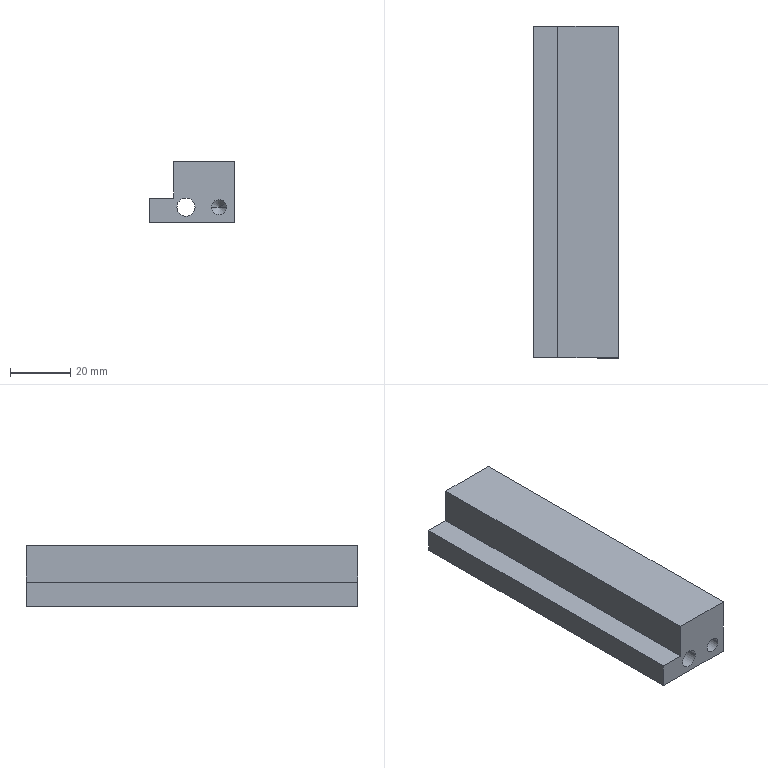Component | SolidWorks | OuterBagSealingCopperBlock-1 | 1 solid | 22 faces | box 28 x 110 x 20 mm | volume 47407 mm3 | cylinder 8 | plane 8 | cone 6 | commonest cylinder face diameters 3.3 x4 5 x2 6 x2
build123d program:
from build123d import *

# Parameters (mm, degrees)
BOSS_EXTRUDE1_DEPTH   = 55
M4_TAPPED_HOLE1_D     = 3.3
M4_TAPPED_HOLE1_DEPTH = 12.1
M4_TAPPED_HOLE1_TIP   = 0.9526
SKETCH4_R             = 3
CUT_EXTRUDE1_DEPTH    = 110
M6_TAPPED_HOLE1_D     = 5
M6_TAPPED_HOLE1_DEPTH = 15
M6_TAPPED_HOLE1_TIP   = 2.5


with BuildPart() as part:
    # Sketch1 → Boss-Extrude1 (new, symmetric)
    with BuildSketch(Plane.XY):
        Polygon((0, 0), (0, 20), (28, 20), (28, 12), (20, 12), (20, 0), align=None)
    extrude(amount=BOSS_EXTRUDE1_DEPTH, both=True)

    # M4 Tapped Hole1
    with Locations(Plane(origin=(0, 10, -25), x_dir=(0, 0, -1), z_dir=(-1, 0, 0))):
        with Locations((0, 0), (-50, 0)):
            Hole(M4_TAPPED_HOLE1_D / 2, depth=M4_TAPPED_HOLE1_DEPTH)
            with Locations((0, 0, -(M4_TAPPED_HOLE1_DEPTH + M4_TAPPED_HOLE1_TIP / 2))):  # 120° drill point
                Cone(0, M4_TAPPED_HOLE1_D / 2, M4_TAPPED_HOLE1_TIP, mode=Mode.SUBTRACT)

    # Sketch4 → Cut-Extrude1 (cut)
    with BuildSketch(Plane.XY.offset(55)):
        with Locations((16, 15)):
            Circle(SKETCH4_R)
    extrude(amount=-CUT_EXTRUDE1_DEPTH, mode=Mode.SUBTRACT)

    # M6 Tapped Hole1
    with Locations(Plane(origin=(5, 15, 55), x_dir=(1, 0, 0), z_dir=(0, 0, 1))):
        with Locations((0, 0)):
            Hole(M6_TAPPED_HOLE1_D / 2, depth=M6_TAPPED_HOLE1_DEPTH)
            with Locations((0, 0, -(M6_TAPPED_HOLE1_DEPTH + M6_TAPPED_HOLE1_TIP / 2))):  # 90° drill point
                Cone(0, M6_TAPPED_HOLE1_D / 2, M6_TAPPED_HOLE1_TIP, mode=Mode.SUBTRACT)


solid = part.part

# Placed as in the assembly
solid = solid.moved(Location((-43.341, 37.185, -31.775), (90, 0, -180)))
STEP:
#1=CARTESIAN_POINT('',(-1.805,-0.1108,-1.842));
#2=VERTEX_POINT('',#1);
#3=CARTESIAN_POINT('',(-2.002,-0.1108,-1.842));
#4=VERTEX_POINT('',#3);
#5=CARTESIAN_POINT('',(-1.903,-0.1108,-1.842));
#6=DIRECTION('',(-0.,-1.,0.));
#7=DIRECTION('',(-1.,0.,0.));
#8=AXIS2_PLACEMENT_3D('',#5,#6,#7);
#9=CIRCLE('',#8,0.09843);
#10=EDGE_CURVE('',#2,#4,#9,.T.);
#11=ORIENTED_EDGE('',*,*,#10,.F.);
#12=CARTESIAN_POINT('',(-1.805,-0.7014,-1.842));
#13=VERTEX_POINT('',#12);
#14=CARTESIAN_POINT('',(-1.805,-0.7014,-1.842));
#15=DIRECTION('',(-0.,-1.,0.));
#16=VECTOR('',#15,39.37);
#17=LINE('',#14,#16);
#18=EDGE_CURVE('',#2,#13,#17,.T.);
#19=ORIENTED_EDGE('',*,*,#18,.T.);
#20=CARTESIAN_POINT('',(-2.002,-0.7014,-1.842));
#21=VERTEX_POINT('',#20);
#22=CARTESIAN_POINT('',(-1.903,-0.7014,-1.842));
#23=DIRECTION('',(-0.,-1.,0.));
#24=DIRECTION('',(-1.,0.,0.));
#25=AXIS2_PLACEMENT_3D('',#22,#23,#24);
#26=CIRCLE('',#25,0.09843);
#27=EDGE_CURVE('',#13,#21,#26,.T.);
#28=ORIENTED_EDGE('',*,*,#27,.T.);
#29=CARTESIAN_POINT('',(-2.002,-0.7014,-1.842));
#30=DIRECTION('',(-0.,-1.,0.));
#31=VECTOR('',#30,39.37);
#32=LINE('',#29,#31);
#33=EDGE_CURVE('',#4,#21,#32,.T.);
#34=ORIENTED_EDGE('',*,*,#33,.F.);
#35=EDGE_LOOP('',(#11,#19,#28,#34));
#36=FACE_OUTER_BOUND('',#35,.T.);
#37=CARTESIAN_POINT('',(-1.903,-0.7014,-1.842));
#38=DIRECTION('',(-0.,-1.,0.));
#39=DIRECTION('',(-1.,0.,0.));
#40=AXIS2_PLACEMENT_3D('',#37,#38,#39);
#41=CYLINDRICAL_SURFACE('',#40,0.09843);
#42=ADVANCED_FACE('',(#36),#41,.F.);
#43=CARTESIAN_POINT('',(-1.903,-0.01239,-1.842));
#44=VERTEX_POINT('',#43);
#45=CARTESIAN_POINT('',(-2.002,-0.1108,-1.842));
#46=DIRECTION('',(-0.7071,-0.7071,0.));
#47=VECTOR('',#46,39.37);
#48=LINE('',#45,#47);
#49=EDGE_CURVE('',#44,#4,#48,.T.);
#50=ORIENTED_EDGE('',*,*,#49,.F.);
#51=CARTESIAN_POINT('',(-1.805,-0.1108,-1.842));
#52=DIRECTION('',(0.7071,-0.7071,-0.));
#53=VECTOR('',#52,39.37);
#54=LINE('',#51,#53);
#55=EDGE_CURVE('',#44,#2,#54,.T.);
#56=ORIENTED_EDGE('',*,*,#55,.T.);
#57=ORIENTED_EDGE('',*,*,#10,.T.);
#58=EDGE_LOOP('',(#50,#56,#57));
#59=FACE_OUTER_BOUND('',#58,.T.);
#60=CARTESIAN_POINT('',(-1.903,-0.1108,-1.842));
#61=DIRECTION('',(-0.,-1.,0.));
#62=DIRECTION('',(-1.,0.,0.));
#63=AXIS2_PLACEMENT_3D('',#60,#61,#62);
#64=CONICAL_SURFACE('',#63,0.09843,0.7854);
#65=ADVANCED_FACE('',(#59),#64,.F.);
#66=CARTESIAN_POINT('',(-2.218,3.629,-1.842));
#67=VERTEX_POINT('',#66);
#68=CARTESIAN_POINT('',(-2.454,3.629,-1.842));
#69=VERTEX_POINT('',#68);
#70=CARTESIAN_POINT('',(-2.336,3.629,-1.842));
#71=DIRECTION('',(-0.,-1.,0.));
#72=DIRECTION('',(-1.,0.,0.));
#73=AXIS2_PLACEMENT_3D('',#70,#71,#72);
#74=CIRCLE('',#73,0.1181);
#75=EDGE_CURVE('',#67,#69,#74,.T.);
#76=ORIENTED_EDGE('',*,*,#75,.F.);
#77=CARTESIAN_POINT('',(-2.218,-0.7014,-1.842));
#78=VERTEX_POINT('',#77);
#79=CARTESIAN_POINT('',(-2.218,3.629,-1.842));
#80=DIRECTION('',(-0.,-1.,0.));
#81=VECTOR('',#80,39.37);
#82=LINE('',#79,#81);
#83=EDGE_CURVE('',#67,#78,#82,.T.);
#84=ORIENTED_EDGE('',*,*,#83,.T.);
#85=CARTESIAN_POINT('',(-2.454,-0.7014,-1.842));
#86=VERTEX_POINT('',#85);
#87=CARTESIAN_POINT('',(-2.336,-0.7014,-1.842));
#88=DIRECTION('',(-0.,-1.,0.));
#89=DIRECTION('',(-1.,0.,0.));
#90=AXIS2_PLACEMENT_3D('',#87,#88,#89);
#91=CIRCLE('',#90,0.1181);
#92=EDGE_CURVE('',#78,#86,#91,.T.);
#93=ORIENTED_EDGE('',*,*,#92,.T.);
#94=CARTESIAN_POINT('',(-2.454,3.629,-1.842));
#95=DIRECTION('',(-0.,-1.,0.));
#96=VECTOR('',#95,39.37);
#97=LINE('',#94,#96);
#98=EDGE_CURVE('',#69,#86,#97,.T.);
#99=ORIENTED_EDGE('',*,*,#98,.F.);
#100=EDGE_LOOP('',(#76,#84,#93,#99));
#101=FACE_OUTER_BOUND('',#100,.T.);
#102=CARTESIAN_POINT('',(-2.336,3.629,-1.842));
#103=DIRECTION('',(-0.,-1.,0.));
#104=DIRECTION('',(-1.,0.,0.));
#105=AXIS2_PLACEMENT_3D('',#102,#103,#104);
#106=CYLINDRICAL_SURFACE('',#105,0.1181);
#107=ADVANCED_FACE('',(#101),#106,.F.);
#108=CARTESIAN_POINT('',(-2.183,2.513,-1.645));
#109=VERTEX_POINT('',#108);
#110=CARTESIAN_POINT('',(-2.183,2.383,-1.645));
#111=VERTEX_POINT('',#110);
#112=CARTESIAN_POINT('',(-2.183,2.448,-1.645));
#113=DIRECTION('',(1.,-0.,-0.));
#114=DIRECTION('',(0.,-1.,0.));
#115=AXIS2_PLACEMENT_3D('',#112,#113,#114);
#116=CIRCLE('',#115,0.06496);
#117=EDGE_CURVE('',#109,#111,#116,.T.);
#118=ORIENTED_EDGE('',*,*,#117,.F.);
#119=CARTESIAN_POINT('',(-1.706,2.513,-1.645));
#120=VERTEX_POINT('',#119);
#121=CARTESIAN_POINT('',(-1.706,2.513,-1.645));
#122=DIRECTION('',(1.,-0.,-0.));
#123=VECTOR('',#122,39.37);
#124=LINE('',#121,#123);
#125=EDGE_CURVE('',#109,#120,#124,.T.);
#126=ORIENTED_EDGE('',*,*,#125,.T.);
#127=CARTESIAN_POINT('',(-1.706,2.383,-1.645));
#128=VERTEX_POINT('',#127);
#129=CARTESIAN_POINT('',(-1.706,2.448,-1.645));
#130=DIRECTION('',(1.,-0.,-0.));
#131=DIRECTION('',(0.,-1.,0.));
#132=AXIS2_PLACEMENT_3D('',#129,#130,#131);
#133=CIRCLE('',#132,0.06496);
#134=EDGE_CURVE('',#120,#128,#133,.T.);
#135=ORIENTED_EDGE('',*,*,#134,.T.);
#136=CARTESIAN_POINT('',(-1.706,2.383,-1.645));
#137=DIRECTION('',(1.,-0.,-0.));
#138=VECTOR('',#137,39.37);
#139=LINE('',#136,#138);
#140=EDGE_CURVE('',#111,#128,#139,.T.);
#141=ORIENTED_EDGE('',*,*,#140,.F.);
#142=EDGE_LOOP('',(#118,#126,#135,#141));
#143=FACE_OUTER_BOUND('',#142,.T.);
#144=CARTESIAN_POINT('',(-1.706,2.448,-1.645));
#145=DIRECTION('',(1.,-0.,-0.));
#146=DIRECTION('',(0.,-1.,0.));
#147=AXIS2_PLACEMENT_3D('',#144,#145,#146);
#148=CYLINDRICAL_SURFACE('',#147,0.06496);
#149=ADVANCED_FACE('',(#143),#148,.F.);
#150=CARTESIAN_POINT('',(-2.22,2.448,-1.645));
#151=VERTEX_POINT('',#150);
#152=CARTESIAN_POINT('',(-2.183,2.383,-1.645));
#153=DIRECTION('',(0.5,-0.866,-0.));
#154=VECTOR('',#153,39.37);
#155=LINE('',#152,#154);
#156=EDGE_CURVE('',#151,#111,#155,.T.);
#157=ORIENTED_EDGE('',*,*,#156,.F.);
#158=CARTESIAN_POINT('',(-2.183,2.513,-1.645));
#159=DIRECTION('',(0.5,0.866,-0.));
#160=VECTOR('',#159,39.37);
#161=LINE('',#158,#160);
#162=EDGE_CURVE('',#151,#109,#161,.T.);
#163=ORIENTED_EDGE('',*,*,#162,.T.);
#164=ORIENTED_EDGE('',*,*,#117,.T.);
#165=EDGE_LOOP('',(#157,#163,#164));
#166=FACE_OUTER_BOUND('',#165,.T.);
#167=CARTESIAN_POINT('',(-2.183,2.448,-1.645));
#168=DIRECTION('',(1.,-0.,-0.));
#169=DIRECTION('',(0.,-1.,0.));
#170=AXIS2_PLACEMENT_3D('',#167,#168,#169);
#171=CONICAL_SURFACE('',#170,0.06496,1.047);
#172=ADVANCED_FACE('',(#166),#171,.F.);
#173=CARTESIAN_POINT('',(-2.183,0.5447,-1.645));
#174=VERTEX_POINT('',#173);
#175=CARTESIAN_POINT('',(-2.183,0.4148,-1.645));
#176=VERTEX_POINT('',#175);
#177=CARTESIAN_POINT('',(-2.183,0.4797,-1.645));
#178=DIRECTION('',(1.,-0.,-0.));
#179=DIRECTION('',(0.,-1.,0.));
#180=AXIS2_PLACEMENT_3D('',#177,#178,#179);
#181=CIRCLE('',#180,0.06496);
#182=EDGE_CURVE('',#174,#176,#181,.T.);
#183=ORIENTED_EDGE('',*,*,#182,.F.);
#184=CARTESIAN_POINT('',(-1.706,0.5447,-1.645));
#185=VERTEX_POINT('',#184);
#186=CARTESIAN_POINT('',(-1.706,0.5447,-1.645));
#187=DIRECTION('',(1.,-0.,-0.));
#188=VECTOR('',#187,39.37);
#189=LINE('',#186,#188);
#190=EDGE_CURVE('',#174,#185,#189,.T.);
#191=ORIENTED_EDGE('',*,*,#190,.T.);
#192=CARTESIAN_POINT('',(-1.706,0.4148,-1.645));
#193=VERTEX_POINT('',#192);
#194=CARTESIAN_POINT('',(-1.706,0.4797,-1.645));
#195=DIRECTION('',(1.,-0.,-0.));
#196=DIRECTION('',(0.,-1.,0.));
#197=AXIS2_PLACEMENT_3D('',#194,#195,#196);
#198=CIRCLE('',#197,0.06496);
#199=EDGE_CURVE('',#185,#193,#198,.T.);
#200=ORIENTED_EDGE('',*,*,#199,.T.);
#201=CARTESIAN_POINT('',(-1.706,0.4148,-1.645));
#202=DIRECTION('',(1.,-0.,-0.));
#203=VECTOR('',#202,39.37);
#204=LINE('',#201,#203);
#205=EDGE_CURVE('',#176,#193,#204,.T.);
#206=ORIENTED_EDGE('',*,*,#205,.F.);
#207=EDGE_LOOP('',(#183,#191,#200,#206));
#208=FACE_OUTER_BOUND('',#207,.T.);
#209=CARTESIAN_POINT('',(-1.706,0.4797,-1.645));
#210=DIRECTION('',(1.,-0.,-0.));
#211=DIRECTION('',(0.,-1.,0.));
#212=AXIS2_PLACEMENT_3D('',#209,#210,#211);
#213=CYLINDRICAL_SURFACE('',#212,0.06496);
#214=ADVANCED_FACE('',(#208),#213,.F.);
#215=CARTESIAN_POINT('',(-2.22,0.4797,-1.645));
#216=VERTEX_POINT('',#215);
#217=CARTESIAN_POINT('',(-2.183,0.4148,-1.645));
#218=DIRECTION('',(0.5,-0.866,-0.));
#219=VECTOR('',#218,39.37);
#220=LINE('',#217,#219);
#221=EDGE_CURVE('',#216,#176,#220,.T.);
#222=ORIENTED_EDGE('',*,*,#221,.F.);
#223=CARTESIAN_POINT('',(-2.183,0.5447,-1.645));
#224=DIRECTION('',(0.5,0.866,-0.));
#225=VECTOR('',#224,39.37);
#226=LINE('',#223,#225);
#227=EDGE_CURVE('',#216,#174,#226,.T.);
#228=ORIENTED_EDGE('',*,*,#227,.T.);
#229=ORIENTED_EDGE('',*,*,#182,.T.);
#230=EDGE_LOOP('',(#222,#228,#229));
#231=FACE_OUTER_BOUND('',#230,.T.);
#232=CARTESIAN_POINT('',(-2.183,0.4797,-1.645));
#233=DIRECTION('',(1.,-0.,-0.));
#234=DIRECTION('',(0.,-1.,0.));
#235=AXIS2_PLACEMENT_3D('',#232,#233,#234);
#236=CONICAL_SURFACE('',#235,0.06496,1.047);
#237=ADVANCED_FACE('',(#231),#236,.F.);
#238=CARTESIAN_POINT('',(-1.706,3.629,-1.251));
#239=VERTEX_POINT('',#238);
#240=CARTESIAN_POINT('',(-2.494,3.629,-1.251));
#241=VERTEX_POINT('',#240);
#242=CARTESIAN_POINT('',(-2.494,3.629,-1.251));
#243=DIRECTION('',(-1.,0.,0.));
#244=VECTOR('',#243,39.37);
#245=LINE('',#242,#244);
#246=EDGE_CURVE('',#239,#241,#245,.T.);
#247=ORIENTED_EDGE('',*,*,#246,.T.);
#248=CARTESIAN_POINT('',(-2.494,-0.7014,-1.251));
#249=VERTEX_POINT('',#248);
#250=CARTESIAN_POINT('',(-2.494,-0.7014,-1.251));
#251=DIRECTION('',(0.,1.,-0.));
#252=VECTOR('',#251,39.37);
#253=LINE('',#250,#252);
#254=EDGE_CURVE('',#249,#241,#253,.T.);
#255=ORIENTED_EDGE('',*,*,#254,.F.);
#256=CARTESIAN_POINT('',(-1.706,-0.7014,-1.251));
#257=VERTEX_POINT('',#256);
#258=CARTESIAN_POINT('',(-2.494,-0.7014,-1.251));
#259=DIRECTION('',(-1.,0.,0.));
#260=VECTOR('',#259,39.37);
#261=LINE('',#258,#260);
#262=EDGE_CURVE('',#257,#249,#261,.T.);
#263=ORIENTED_EDGE('',*,*,#262,.F.);
#264=CARTESIAN_POINT('',(-1.706,-0.7014,-1.251));
#265=DIRECTION('',(0.,1.,-0.));
#266=VECTOR('',#265,39.37);
#267=LINE('',#264,#266);
#268=EDGE_CURVE('',#257,#239,#267,.T.);
#269=ORIENTED_EDGE('',*,*,#268,.T.);
#270=EDGE_LOOP('',(#247,#255,#263,#269));
#271=FACE_OUTER_BOUND('',#270,.T.);
#272=CARTESIAN_POINT('',(-2.494,-0.7014,-1.251));
#273=DIRECTION('',(-0.,-0.,-1.));
#274=DIRECTION('',(-0.,-1.,0.));
#275=AXIS2_PLACEMENT_3D('',#272,#273,#274);
#276=PLANE('',#275);
#277=ADVANCED_FACE('',(#271),#276,.F.);
#278=CARTESIAN_POINT('',(-2.494,3.629,-1.723));
#279=VERTEX_POINT('',#278);
#280=CARTESIAN_POINT('',(-2.494,3.629,-1.723));
#281=DIRECTION('',(-0.,-0.,-1.));
#282=VECTOR('',#281,39.37);
#283=LINE('',#280,#282);
#284=EDGE_CURVE('',#241,#279,#283,.T.);
#285=ORIENTED_EDGE('',*,*,#284,.T.);
#286=CARTESIAN_POINT('',(-2.494,-0.7014,-1.723));
#287=VERTEX_POINT('',#286);
#288=CARTESIAN_POINT('',(-2.494,-0.7014,-1.723));
#289=DIRECTION('',(0.,1.,-0.));
#290=VECTOR('',#289,39.37);
#291=LINE('',#288,#290);
#292=EDGE_CURVE('',#287,#279,#291,.T.);
#293=ORIENTED_EDGE('',*,*,#292,.F.);
#294=CARTESIAN_POINT('',(-2.494,-0.7014,-1.723));
#295=DIRECTION('',(-0.,-0.,-1.));
#296=VECTOR('',#295,39.37);
#297=LINE('',#294,#296);
#298=EDGE_CURVE('',#249,#287,#297,.T.);
#299=ORIENTED_EDGE('',*,*,#298,.F.);
#300=ORIENTED_EDGE('',*,*,#254,.T.);
#301=EDGE_LOOP('',(#285,#293,#299,#300));
#302=FACE_OUTER_BOUND('',#301,.T.);
#303=CARTESIAN_POINT('',(-2.494,-0.7014,-1.723));
#304=DIRECTION('',(1.,-0.,-0.));
#305=DIRECTION('',(-0.,-1.,0.));
#306=AXIS2_PLACEMENT_3D('',#303,#304,#305);
#307=PLANE('',#306);
#308=ADVANCED_FACE('',(#302),#307,.F.);
#309=CARTESIAN_POINT('',(-2.809,3.629,-1.723));
#310=VERTEX_POINT('',#309);
#311=CARTESIAN_POINT('',(-2.809,3.629,-1.723));
#312=DIRECTION('',(-1.,0.,0.));
#313=VECTOR('',#312,39.37);
#314=LINE('',#311,#313);
#315=EDGE_CURVE('',#279,#310,#314,.T.);
#316=ORIENTED_EDGE('',*,*,#315,.T.);
#317=CARTESIAN_POINT('',(-2.809,-0.7014,-1.723));
#318=VERTEX_POINT('',#317);
#319=CARTESIAN_POINT('',(-2.809,-0.7014,-1.723));
#320=DIRECTION('',(0.,1.,-0.));
#321=VECTOR('',#320,39.37);
#322=LINE('',#319,#321);
#323=EDGE_CURVE('',#318,#310,#322,.T.);
#324=ORIENTED_EDGE('',*,*,#323,.F.);
#325=CARTESIAN_POINT('',(-2.809,-0.7014,-1.723));
#326=DIRECTION('',(-1.,0.,0.));
#327=VECTOR('',#326,39.37);
#328=LINE('',#325,#327);
#329=EDGE_CURVE('',#287,#318,#328,.T.);
#330=ORIENTED_EDGE('',*,*,#329,.F.);
#331=ORIENTED_EDGE('',*,*,#292,.T.);
#332=EDGE_LOOP('',(#316,#324,#330,#331));
#333=FACE_OUTER_BOUND('',#332,.T.);
#334=CARTESIAN_POINT('',(-2.809,-0.7014,-1.723));
#335=DIRECTION('',(-0.,-0.,-1.));
#336=DIRECTION('',(1.,-0.,-0.));
#337=AXIS2_PLACEMENT_3D('',#334,#335,#336);
#338=PLANE('',#337);
#339=ADVANCED_FACE('',(#333),#338,.F.);
#340=CARTESIAN_POINT('',(-2.809,3.629,-2.038));
#341=VERTEX_POINT('',#340);
#342=CARTESIAN_POINT('',(-2.809,3.629,-2.038));
#343=DIRECTION('',(-0.,-0.,-1.));
#344=VECTOR('',#343,39.37);
#345=LINE('',#342,#344);
#346=EDGE_CURVE('',#310,#341,#345,.T.);
#347=ORIENTED_EDGE('',*,*,#346,.T.);
#348=CARTESIAN_POINT('',(-2.809,-0.7014,-2.038));
#349=VERTEX_POINT('',#348);
#350=CARTESIAN_POINT('',(-2.809,-0.7014,-2.038));
#351=DIRECTION('',(0.,1.,-0.));
#352=VECTOR('',#351,39.37);
#353=LINE('',#350,#352);
#354=EDGE_CURVE('',#349,#341,#353,.T.);
#355=ORIENTED_EDGE('',*,*,#354,.F.);
#356=CARTESIAN_POINT('',(-2.809,-0.7014,-2.038));
#357=DIRECTION('',(-0.,-0.,-1.));
#358=VECTOR('',#357,39.37);
#359=LINE('',#356,#358);
#360=EDGE_CURVE('',#318,#349,#359,.T.);
#361=ORIENTED_EDGE('',*,*,#360,.F.);
#362=ORIENTED_EDGE('',*,*,#323,.T.);
#363=EDGE_LOOP('',(#347,#355,#361,#362));
#364=FACE_OUTER_BOUND('',#363,.T.);
#365=CARTESIAN_POINT('',(-2.809,-0.7014,-2.038));
#366=DIRECTION('',(1.,-0.,-0.));
#367=DIRECTION('',(0.,0.,1.));
#368=AXIS2_PLACEMENT_3D('',#365,#366,#367);
#369=PLANE('',#368);
#370=ADVANCED_FACE('',(#364),#369,.F.);
#371=CARTESIAN_POINT('',(-1.706,3.629,-2.038));
#372=VERTEX_POINT('',#371);
#373=CARTESIAN_POINT('',(-1.706,3.629,-2.038));
#374=DIRECTION('',(1.,-0.,-0.));
#375=VECTOR('',#374,39.37);
#376=LINE('',#373,#375);
#377=EDGE_CURVE('',#341,#372,#376,.T.);
#378=ORIENTED_EDGE('',*,*,#377,.T.);
#379=CARTESIAN_POINT('',(-1.706,-0.7014,-2.038));
#380=VERTEX_POINT('',#379);
#381=CARTESIAN_POINT('',(-1.706,-0.7014,-2.038));
#382=DIRECTION('',(0.,1.,-0.));
#383=VECTOR('',#382,39.37);
#384=LINE('',#381,#383);
#385=EDGE_CURVE('',#380,#372,#384,.T.);
#386=ORIENTED_EDGE('',*,*,#385,.F.);
#387=CARTESIAN_POINT('',(-1.706,-0.7014,-2.038));
#388=DIRECTION('',(1.,-0.,-0.));
#389=VECTOR('',#388,39.37);
#390=LINE('',#387,#389);
#391=EDGE_CURVE('',#349,#380,#390,.T.);
#392=ORIENTED_EDGE('',*,*,#391,.F.);
#393=ORIENTED_EDGE('',*,*,#354,.T.);
#394=EDGE_LOOP('',(#378,#386,#392,#393));
#395=FACE_OUTER_BOUND('',#394,.T.);
#396=CARTESIAN_POINT('',(-1.706,-0.7014,-2.038));
#397=DIRECTION('',(0.,0.,1.));
#398=DIRECTION('',(0.,1.,-0.));
#399=AXIS2_PLACEMENT_3D('',#396,#397,#398);
#400=PLANE('',#399);
#401=ADVANCED_FACE('',(#395),#400,.F.);
#402=CARTESIAN_POINT('',(-1.706,2.448,-1.645));
#403=DIRECTION('',(1.,-0.,-0.));
#404=DIRECTION('',(0.,-1.,0.));
#405=AXIS2_PLACEMENT_3D('',#402,#403,#404);
#406=CIRCLE('',#405,0.06496);
#407=EDGE_CURVE('',#128,#120,#406,.T.);
#408=ORIENTED_EDGE('',*,*,#407,.F.);
#409=ORIENTED_EDGE('',*,*,#134,.F.);
#410=EDGE_LOOP('',(#408,#409));
#411=FACE_BOUND('',#410,.T.);
#412=CARTESIAN_POINT('',(-1.706,0.4797,-1.645));
#413=DIRECTION('',(1.,-0.,-0.));
#414=DIRECTION('',(0.,-1.,0.));
#415=AXIS2_PLACEMENT_3D('',#412,#413,#414);
#416=CIRCLE('',#415,0.06496);
#417=EDGE_CURVE('',#193,#185,#416,.T.);
#418=ORIENTED_EDGE('',*,*,#417,.F.);
#419=ORIENTED_EDGE('',*,*,#199,.F.);
#420=EDGE_LOOP('',(#418,#419));
#421=FACE_BOUND('',#420,.T.);
#422=CARTESIAN_POINT('',(-1.706,3.629,-1.251));
#423=DIRECTION('',(0.,0.,1.));
#424=VECTOR('',#423,39.37);
#425=LINE('',#422,#424);
#426=EDGE_CURVE('',#372,#239,#425,.T.);
#427=ORIENTED_EDGE('',*,*,#426,.T.);
#428=ORIENTED_EDGE('',*,*,#268,.F.);
#429=CARTESIAN_POINT('',(-1.706,-0.7014,-1.251));
#430=DIRECTION('',(0.,0.,1.));
#431=VECTOR('',#430,39.37);
#432=LINE('',#429,#431);
#433=EDGE_CURVE('',#380,#257,#432,.T.);
#434=ORIENTED_EDGE('',*,*,#433,.F.);
#435=ORIENTED_EDGE('',*,*,#385,.T.);
#436=EDGE_LOOP('',(#427,#428,#434,#435));
#437=FACE_OUTER_BOUND('',#436,.T.);
#438=CARTESIAN_POINT('',(-1.706,-0.7014,-1.251));
#439=DIRECTION('',(-1.,0.,0.));
#440=DIRECTION('',(0.,1.,-0.));
#441=AXIS2_PLACEMENT_3D('',#438,#439,#440);
#442=PLANE('',#441);
#443=ADVANCED_FACE('',(#411,#421,#437),#442,.F.);
#444=CARTESIAN_POINT('',(-1.903,-0.7014,-1.842));
#445=DIRECTION('',(-0.,-1.,0.));
#446=DIRECTION('',(-1.,0.,0.));
#447=AXIS2_PLACEMENT_3D('',#444,#445,#446);
#448=CIRCLE('',#447,0.09843);
#449=EDGE_CURVE('',#21,#13,#448,.T.);
#450=ORIENTED_EDGE('',*,*,#449,.F.);
#451=ORIENTED_EDGE('',*,*,#27,.F.);
#452=EDGE_LOOP('',(#450,#451));
#453=FACE_BOUND('',#452,.T.);
#454=CARTESIAN_POINT('',(-2.336,-0.7014,-1.842));
#455=DIRECTION('',(-0.,-1.,0.));
#456=DIRECTION('',(-1.,0.,0.));
#457=AXIS2_PLACEMENT_3D('',#454,#455,#456);
#458=CIRCLE('',#457,0.1181);
#459=EDGE_CURVE('',#86,#78,#458,.T.);
#460=ORIENTED_EDGE('',*,*,#459,.F.);
#461=ORIENTED_EDGE('',*,*,#92,.F.);
#462=EDGE_LOOP('',(#460,#461));
#463=FACE_BOUND('',#462,.T.);
#464=ORIENTED_EDGE('',*,*,#262,.T.);
#465=ORIENTED_EDGE('',*,*,#298,.T.);
#466=ORIENTED_EDGE('',*,*,#329,.T.);
#467=ORIENTED_EDGE('',*,*,#360,.T.);
#468=ORIENTED_EDGE('',*,*,#391,.T.);
#469=ORIENTED_EDGE('',*,*,#433,.T.);
#470=EDGE_LOOP('',(#464,#465,#466,#467,#468,#469));
#471=FACE_OUTER_BOUND('',#470,.T.);
#472=CARTESIAN_POINT('',(-1.706,-0.7014,-1.251));
#473=DIRECTION('',(0.,1.,-0.));
#474=DIRECTION('',(1.,-0.,-0.));
#475=AXIS2_PLACEMENT_3D('',#472,#473,#474);
#476=PLANE('',#475);
#477=ADVANCED_FACE('',(#453,#463,#471),#476,.F.);
#478=CARTESIAN_POINT('',(-2.336,3.629,-1.842));
#479=DIRECTION('',(-0.,-1.,0.));
#480=DIRECTION('',(-1.,0.,0.));
#481=AXIS2_PLACEMENT_3D('',#478,#479,#480);
#482=CIRCLE('',#481,0.1181);
#483=EDGE_CURVE('',#69,#67,#482,.T.);
#484=ORIENTED_EDGE('',*,*,#483,.T.);
#485=ORIENTED_EDGE('',*,*,#75,.T.);
#486=EDGE_LOOP('',(#484,#485));
#487=FACE_BOUND('',#486,.T.);
#488=ORIENTED_EDGE('',*,*,#246,.F.);
#489=ORIENTED_EDGE('',*,*,#426,.F.);
#490=ORIENTED_EDGE('',*,*,#377,.F.);
#491=ORIENTED_EDGE('',*,*,#346,.F.);
#492=ORIENTED_EDGE('',*,*,#315,.F.);
#493=ORIENTED_EDGE('',*,*,#284,.F.);
#494=EDGE_LOOP('',(#488,#489,#490,#491,#492,#493));
#495=FACE_OUTER_BOUND('',#494,.T.);
#496=CARTESIAN_POINT('',(-1.706,3.629,-1.251));
#497=DIRECTION('',(0.,1.,-0.));
#498=DIRECTION('',(1.,-0.,-0.));
#499=AXIS2_PLACEMENT_3D('',#496,#497,#498);
#500=PLANE('',#499);
#501=ADVANCED_FACE('',(#487,#495),#500,.T.);
#502=ORIENTED_EDGE('',*,*,#227,.F.);
#503=ORIENTED_EDGE('',*,*,#221,.T.);
#504=CARTESIAN_POINT('',(-2.183,0.4797,-1.645));
#505=DIRECTION('',(1.,-0.,-0.));
#506=DIRECTION('',(0.,-1.,0.));
#507=AXIS2_PLACEMENT_3D('',#504,#505,#506);
#508=CIRCLE('',#507,0.06496);
#509=EDGE_CURVE('',#176,#174,#508,.T.);
#510=ORIENTED_EDGE('',*,*,#509,.T.);
#511=EDGE_LOOP('',(#502,#503,#510));
#512=FACE_OUTER_BOUND('',#511,.T.);
#513=CARTESIAN_POINT('',(-2.183,0.4797,-1.645));
#514=DIRECTION('',(1.,-0.,-0.));
#515=DIRECTION('',(0.,-1.,0.));
#516=AXIS2_PLACEMENT_3D('',#513,#514,#515);
#517=CONICAL_SURFACE('',#516,0.06496,1.047);
#518=ADVANCED_FACE('',(#512),#517,.F.);
#519=ORIENTED_EDGE('',*,*,#190,.F.);
#520=ORIENTED_EDGE('',*,*,#509,.F.);
#521=ORIENTED_EDGE('',*,*,#205,.T.);
#522=ORIENTED_EDGE('',*,*,#417,.T.);
#523=EDGE_LOOP('',(#519,#520,#521,#522));
#524=FACE_OUTER_BOUND('',#523,.T.);
#525=CARTESIAN_POINT('',(-1.706,0.4797,-1.645));
#526=DIRECTION('',(1.,-0.,-0.));
#527=DIRECTION('',(0.,-1.,0.));
#528=AXIS2_PLACEMENT_3D('',#525,#526,#527);
#529=CYLINDRICAL_SURFACE('',#528,0.06496);
#530=ADVANCED_FACE('',(#524),#529,.F.);
#531=ORIENTED_EDGE('',*,*,#162,.F.);
#532=ORIENTED_EDGE('',*,*,#156,.T.);
#533=CARTESIAN_POINT('',(-2.183,2.448,-1.645));
#534=DIRECTION('',(1.,-0.,-0.));
#535=DIRECTION('',(0.,-1.,0.));
#536=AXIS2_PLACEMENT_3D('',#533,#534,#535);
#537=CIRCLE('',#536,0.06496);
#538=EDGE_CURVE('',#111,#109,#537,.T.);
#539=ORIENTED_EDGE('',*,*,#538,.T.);
#540=EDGE_LOOP('',(#531,#532,#539));
#541=FACE_OUTER_BOUND('',#540,.T.);
#542=CARTESIAN_POINT('',(-2.183,2.448,-1.645));
#543=DIRECTION('',(1.,-0.,-0.));
#544=DIRECTION('',(0.,-1.,0.));
#545=AXIS2_PLACEMENT_3D('',#542,#543,#544);
#546=CONICAL_SURFACE('',#545,0.06496,1.047);
#547=ADVANCED_FACE('',(#541),#546,.F.);
#548=ORIENTED_EDGE('',*,*,#125,.F.);
#549=ORIENTED_EDGE('',*,*,#538,.F.);
#550=ORIENTED_EDGE('',*,*,#140,.T.);
#551=ORIENTED_EDGE('',*,*,#407,.T.);
#552=EDGE_LOOP('',(#548,#549,#550,#551));
#553=FACE_OUTER_BOUND('',#552,.T.);
#554=CARTESIAN_POINT('',(-1.706,2.448,-1.645));
#555=DIRECTION('',(1.,-0.,-0.));
#556=DIRECTION('',(0.,-1.,0.));
#557=AXIS2_PLACEMENT_3D('',#554,#555,#556);
#558=CYLINDRICAL_SURFACE('',#557,0.06496);
#559=ADVANCED_FACE('',(#553),#558,.F.);
#560=ORIENTED_EDGE('',*,*,#83,.F.);
#561=ORIENTED_EDGE('',*,*,#483,.F.);
#562=ORIENTED_EDGE('',*,*,#98,.T.);
#563=ORIENTED_EDGE('',*,*,#459,.T.);
#564=EDGE_LOOP('',(#560,#561,#562,#563));
#565=FACE_OUTER_BOUND('',#564,.T.);
#566=CARTESIAN_POINT('',(-2.336,3.629,-1.842));
#567=DIRECTION('',(-0.,-1.,0.));
#568=DIRECTION('',(-1.,0.,0.));
#569=AXIS2_PLACEMENT_3D('',#566,#567,#568);
#570=CYLINDRICAL_SURFACE('',#569,0.1181);
#571=ADVANCED_FACE('',(#565),#570,.F.);
#572=ORIENTED_EDGE('',*,*,#55,.F.);
#573=ORIENTED_EDGE('',*,*,#49,.T.);
#574=CARTESIAN_POINT('',(-1.903,-0.1108,-1.842));
#575=DIRECTION('',(-0.,-1.,0.));
#576=DIRECTION('',(-1.,0.,0.));
#577=AXIS2_PLACEMENT_3D('',#574,#575,#576);
#578=CIRCLE('',#577,0.09843);
#579=EDGE_CURVE('',#4,#2,#578,.T.);
#580=ORIENTED_EDGE('',*,*,#579,.T.);
#581=EDGE_LOOP('',(#572,#573,#580));
#582=FACE_OUTER_BOUND('',#581,.T.);
#583=CARTESIAN_POINT('',(-1.903,-0.1108,-1.842));
#584=DIRECTION('',(-0.,-1.,0.));
#585=DIRECTION('',(-1.,0.,0.));
#586=AXIS2_PLACEMENT_3D('',#583,#584,#585);
#587=CONICAL_SURFACE('',#586,0.09843,0.7854);
#588=ADVANCED_FACE('',(#582),#587,.F.);
#589=ORIENTED_EDGE('',*,*,#18,.F.);
#590=ORIENTED_EDGE('',*,*,#579,.F.);
#591=ORIENTED_EDGE('',*,*,#33,.T.);
#592=ORIENTED_EDGE('',*,*,#449,.T.);
#593=EDGE_LOOP('',(#589,#590,#591,#592));
#594=FACE_OUTER_BOUND('',#593,.T.);
#595=CARTESIAN_POINT('',(-1.903,-0.7014,-1.842));
#596=DIRECTION('',(-0.,-1.,0.));
#597=DIRECTION('',(-1.,0.,0.));
#598=AXIS2_PLACEMENT_3D('',#595,#596,#597);
#599=CYLINDRICAL_SURFACE('',#598,0.09843);
#600=ADVANCED_FACE('',(#594),#599,.F.);
#601=CLOSED_SHELL('',(#42,#65,#107,#149,#172,#214,#237,#277,#308,#339,#370,#401,#443,#477,#501,#518,#530,#547,#559,#571,#588,#600));
#602=MANIFOLD_SOLID_BREP('',#601);
#603=CARTESIAN_POINT('',(0.,0.,0.));
#604=DIRECTION('',(0.,0.,1.));
#605=DIRECTION('',(1.,0.,0.));
#606=AXIS2_PLACEMENT_3D('',#603,#604,#605);
#607=(LENGTH_UNIT()NAMED_UNIT(*)SI_UNIT($,.METRE.));
#608=LENGTH_MEASURE_WITH_UNIT(LENGTH_MEASURE(0.0254),#607);
#609=DIMENSIONAL_EXPONENTS(1.,0.,0.,0.,0.,0.,0.);
#610=(CONVERSION_BASED_UNIT('',#608)LENGTH_UNIT()NAMED_UNIT(#609));
#611=UNCERTAINTY_MEASURE_WITH_UNIT(LENGTH_MEASURE(0.00001),#610,'','');
#612=(NAMED_UNIT(*)PLANE_ANGLE_UNIT()SI_UNIT($,.RADIAN.));
#613=(NAMED_UNIT(*)SI_UNIT($,.STERADIAN.)SOLID_ANGLE_UNIT());
#614=(GEOMETRIC_REPRESENTATION_CONTEXT(3)GLOBAL_UNCERTAINTY_ASSIGNED_CONTEXT((#611))GLOBAL_UNIT_ASSIGNED_CONTEXT((#610,#612,#613))REPRESENTATION_CONTEXT('',''));
#615=ADVANCED_BREP_SHAPE_REPRESENTATION('',(#602,#606),#614);
#616=COLOUR_RGB('',0.7922,0.8196,0.9333);
#617=FILL_AREA_STYLE_COLOUR('',#616);
#618=FILL_AREA_STYLE('',(#617));
#619=SURFACE_STYLE_FILL_AREA(#618);
#620=SURFACE_SIDE_STYLE('',(#619));
#621=SURFACE_STYLE_USAGE(.BOTH.,#620);
#622=PRESENTATION_STYLE_ASSIGNMENT((#621));
#623=STYLED_ITEM('',(#622),#602);
#624=PRESENTATION_LAYER_ASSIGNMENT('','',(#623));
#625=(LENGTH_UNIT()NAMED_UNIT(*)SI_UNIT($,.METRE.));
#626=LENGTH_MEASURE_WITH_UNIT(LENGTH_MEASURE(0.0254),#625);
#627=DIMENSIONAL_EXPONENTS(1.,0.,0.,0.,0.,0.,0.);
#628=(CONVERSION_BASED_UNIT('',#626)LENGTH_UNIT()NAMED_UNIT(#627));
#629=UNCERTAINTY_MEASURE_WITH_UNIT(LENGTH_MEASURE(0.00001),#628,'','');
#630=(NAMED_UNIT(*)PLANE_ANGLE_UNIT()SI_UNIT($,.RADIAN.));
#631=(NAMED_UNIT(*)SI_UNIT($,.STERADIAN.)SOLID_ANGLE_UNIT());
#632=(GEOMETRIC_REPRESENTATION_CONTEXT(3)GLOBAL_UNCERTAINTY_ASSIGNED_CONTEXT((#629))GLOBAL_UNIT_ASSIGNED_CONTEXT((#628,#630,#631))REPRESENTATION_CONTEXT('',''));
#633=MECHANICAL_DESIGN_GEOMETRIC_PRESENTATION_REPRESENTATION('',(#623),#632);